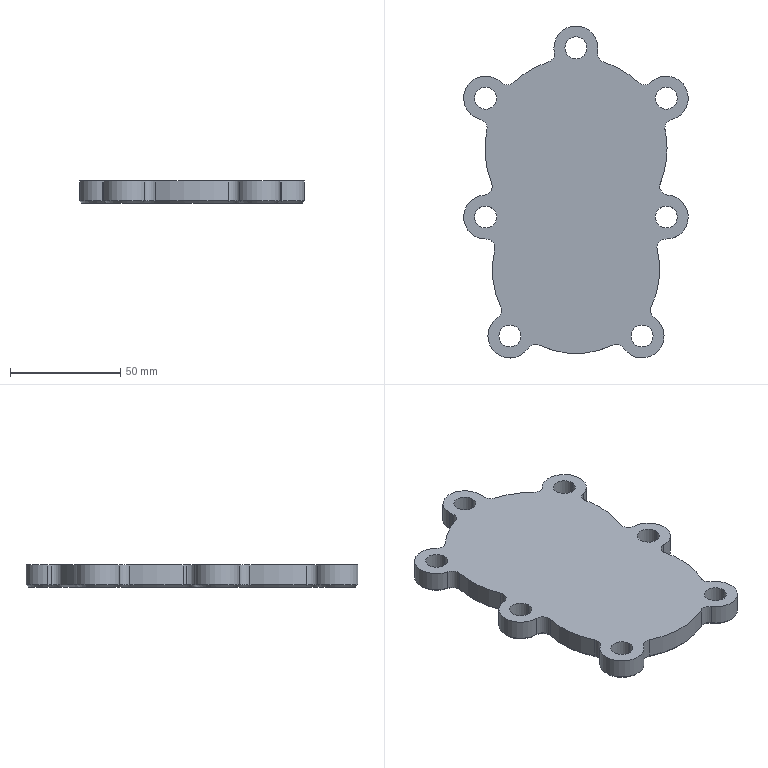Component | SolidWorks | PumpBodyPartTwo-1 | 1 solid | 96 faces | box 102 x 150.83 x 10 mm | volume 103839 mm3 | cylinder 54 | cone 40 | plane 2 | commonest cylinder face diameters 8 x19 10 x14 20 x12 82.709 x5 76 x4
build123d program:
from build123d import *

# Parameters (mm, degrees)
SKETCH1_R           = 5
BOSS_EXTRUDE2_DEPTH = 10
FILLET1_R           = 4
CHAMFER1_SIZE       = 1


with BuildPart() as part:
    # Sketch1 → Boss-Extrude2 (new body)
    with BuildSketch(Plane.XY):
        with BuildLine():
            ThreePointArc((34.106, -38.244), (50.142, -35.052), (41.738, -21.027))
            ThreePointArc((41.738, -21.027), (38.635, -19.149), (38.326, -15.535))
            ThreePointArc((38.326, -15.535), (41.335, -1.265), (39.204, 13.163))
            ThreePointArc((39.204, 13.163), (49.721, 27.893), (31.669, 26.595))
            ThreePointArc((31.669, 26.595), (21.228, 35.491), (8.452, 40.482))
            ThreePointArc((8.452, 40.482), (0, 55.827), (-8.452, 40.482))
            ThreePointArc((-8.452, 40.482), (-21.228, 35.491), (-31.669, 26.595))
            ThreePointArc((-31.669, 26.595), (-49.721, 27.893), (-39.204, 13.163))
            ThreePointArc((-39.204, 13.163), (-41.335, -1.265), (-38.326, -15.535))
            ThreePointArc((-38.326, -15.535), (-38.635, -19.149), (-41.738, -21.027))
            ThreePointArc((-41.738, -21.027), (-50.142, -35.052), (-34.106, -38.244))
            ThreePointArc((-34.106, -38.244), (-37.948, -56.993), (-32.163, -75.237))
            ThreePointArc((-32.163, -75.237), (-37.071, -92.071), (-20.237, -87.163))
            ThreePointArc((-20.237, -87.163), (0, -93), (20.237, -87.163))
            ThreePointArc((20.237, -87.163), (37.071, -92.071), (32.163, -75.237))
            ThreePointArc((32.163, -75.237), (37.948, -56.993), (34.106, -38.244))
        make_face()
        with Locations((-30, -85)):
            Circle(SKETCH1_R, mode=Mode.SUBTRACT)
        with Locations((0, 45.827)):
            Circle(SKETCH1_R, mode=Mode.SUBTRACT)
        with Locations((30, -85)):
            Circle(SKETCH1_R, mode=Mode.SUBTRACT)
        with Locations((41, -31)):
            Circle(SKETCH1_R, mode=Mode.SUBTRACT)
        with Locations((41, 23)):
            Circle(SKETCH1_R, mode=Mode.SUBTRACT)
        with Locations((-41, 23)):
            Circle(SKETCH1_R, mode=Mode.SUBTRACT)
        with Locations((-41, -31)):
            Circle(SKETCH1_R, mode=Mode.SUBTRACT)
    extrude(amount=BOSS_EXTRUDE2_DEPTH)

    # Fillet1
    fillet1_edges = [part.edges().sort_by_distance(p)[0] for p in [
        (8.452, 40.482, 5),
        (31.669, 26.595, 5),
        (39.204, 13.163, 5),
        (34.106, -38.244, 5),
        (32.163, -75.237, 5),
        (20.237, -87.163, 5),
        (-20.237, -87.163, 5),
        (-32.163, -75.237, 5),
        (-34.106, -38.244, 5),
        (-39.204, 13.163, 5),
        (-31.669, 26.595, 5),
        (-8.452, 40.482, 5),
    ]]
    fillet(fillet1_edges, radius=FILLET1_R)

    # Chamfer1
    chamfer1_edges = [part.edges().sort_by_distance(p)[0] for p in [
        (31.203, 28.958, 10),
        (40.977, 11.534, 10),
        (37.663, -42.506, 10),
        (33.915, -74.405, 10),
        (19.405, -88.915, 10),
        (-19.405, -88.915, 10),
        (-33.915, -74.405, 10),
        (-40.977, 11.534, 10),
        (-31.203, 28.958, 10),
        (-10.319, 41.17, 10),
        (-37.663, -42.506, 10),
        (-38.635, -19.149, 10),
        (-50.99, -31.443, 10),
        (50.99, -31.443, 10),
        (38.635, -19.149, 10),
        (0, 55.827, 10),
        (21.004, 35.624, 10),
        (41.195, -3.636, 10),
        (49.721, 27.893, 10),
        (37.787, -59.019, 10),
        (37.071, -92.071, 10),
        (0, -93, 10),
        (-37.071, -92.071, 10),
        (-37.787, -59.019, 10),
        (-41.195, -3.636, 10),
        (-49.721, 27.893, 10),
        (-21.004, 35.624, 10),
        (10.319, 41.17, 10),
    ]]
    chamfer(chamfer1_edges, length=CHAMFER1_SIZE)


solid = part.part

# Placed as in the assembly
solid = solid.moved(Location((-80.719, 26.515, 109.5), (-180, 0, 180)))